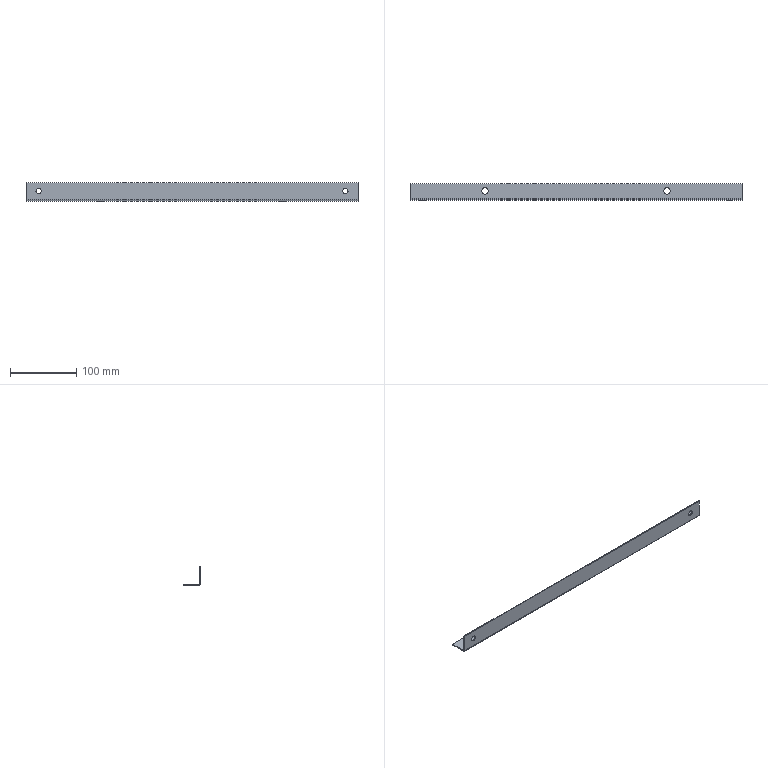Component | SolidWorks | ALK K_EBENT-3 | 1 solid | 22 faces | box 500 x 25.5 x 28.5 mm | volume 38510 mm3 | plane 12 | cylinder 10 | commonest cylinder face diameters 8 x4 10 x4 1.473 x1 4.473 x1
STEP:
#1=CARTESIAN_POINT('',(12.868,0.4007,-13.525));
#2=VERTEX_POINT('',#1);
#3=CARTESIAN_POINT('',(12.553,0.4007,-13.525));
#4=VERTEX_POINT('',#3);
#5=CARTESIAN_POINT('',(12.711,0.4007,-13.525));
#6=DIRECTION('',(0.,1.,0.));
#7=DIRECTION('',(-1.,0.,0.));
#8=AXIS2_PLACEMENT_3D('',#5,#6,#7);
#9=CIRCLE('',#8,0.1575);
#10=EDGE_CURVE('',#2,#4,#9,.T.);
#11=ORIENTED_EDGE('',*,*,#10,.F.);
#12=CARTESIAN_POINT('',(12.868,0.4597,-13.525));
#13=VERTEX_POINT('',#12);
#14=CARTESIAN_POINT('',(12.868,0.06603,-13.525));
#15=DIRECTION('',(0.,1.,0.));
#16=VECTOR('',#15,39.37);
#17=LINE('',#14,#16);
#18=EDGE_CURVE('',#2,#13,#17,.T.);
#19=ORIENTED_EDGE('',*,*,#18,.T.);
#20=CARTESIAN_POINT('',(12.553,0.4597,-13.525));
#21=VERTEX_POINT('',#20);
#22=CARTESIAN_POINT('',(12.711,0.4597,-13.525));
#23=DIRECTION('',(0.,1.,0.));
#24=DIRECTION('',(-1.,0.,0.));
#25=AXIS2_PLACEMENT_3D('',#22,#23,#24);
#26=CIRCLE('',#25,0.1575);
#27=EDGE_CURVE('',#13,#21,#26,.T.);
#28=ORIENTED_EDGE('',*,*,#27,.T.);
#29=CARTESIAN_POINT('',(12.553,0.06603,-13.525));
#30=DIRECTION('',(0.,1.,0.));
#31=VECTOR('',#30,39.37);
#32=LINE('',#29,#31);
#33=EDGE_CURVE('',#4,#21,#32,.T.);
#34=ORIENTED_EDGE('',*,*,#33,.F.);
#35=EDGE_LOOP('',(#11,#19,#28,#34));
#36=FACE_OUTER_BOUND('',#35,.T.);
#37=CARTESIAN_POINT('',(12.711,0.06603,-13.525));
#38=DIRECTION('',(0.,1.,0.));
#39=DIRECTION('',(-1.,0.,0.));
#40=AXIS2_PLACEMENT_3D('',#37,#38,#39);
#41=CYLINDRICAL_SURFACE('',#40,0.1575);
#42=ADVANCED_FACE('',(#36),#41,.F.);
#43=CARTESIAN_POINT('',(-5.321,0.4007,-13.525));
#44=VERTEX_POINT('',#43);
#45=CARTESIAN_POINT('',(-5.636,0.4007,-13.525));
#46=VERTEX_POINT('',#45);
#47=CARTESIAN_POINT('',(-5.478,0.4007,-13.525));
#48=DIRECTION('',(0.,1.,0.));
#49=DIRECTION('',(-1.,0.,0.));
#50=AXIS2_PLACEMENT_3D('',#47,#48,#49);
#51=CIRCLE('',#50,0.1575);
#52=EDGE_CURVE('',#44,#46,#51,.T.);
#53=ORIENTED_EDGE('',*,*,#52,.F.);
#54=CARTESIAN_POINT('',(-5.321,0.4597,-13.525));
#55=VERTEX_POINT('',#54);
#56=CARTESIAN_POINT('',(-5.321,0.06603,-13.525));
#57=DIRECTION('',(0.,1.,0.));
#58=VECTOR('',#57,39.37);
#59=LINE('',#56,#58);
#60=EDGE_CURVE('',#44,#55,#59,.T.);
#61=ORIENTED_EDGE('',*,*,#60,.T.);
#62=CARTESIAN_POINT('',(-5.636,0.4597,-13.525));
#63=VERTEX_POINT('',#62);
#64=CARTESIAN_POINT('',(-5.478,0.4597,-13.525));
#65=DIRECTION('',(0.,1.,0.));
#66=DIRECTION('',(-1.,0.,0.));
#67=AXIS2_PLACEMENT_3D('',#64,#65,#66);
#68=CIRCLE('',#67,0.1575);
#69=EDGE_CURVE('',#55,#63,#68,.T.);
#70=ORIENTED_EDGE('',*,*,#69,.T.);
#71=CARTESIAN_POINT('',(-5.636,0.06603,-13.525));
#72=DIRECTION('',(0.,1.,0.));
#73=VECTOR('',#72,39.37);
#74=LINE('',#71,#73);
#75=EDGE_CURVE('',#46,#63,#74,.T.);
#76=ORIENTED_EDGE('',*,*,#75,.F.);
#77=EDGE_LOOP('',(#53,#61,#70,#76));
#78=FACE_OUTER_BOUND('',#77,.T.);
#79=CARTESIAN_POINT('',(-5.478,0.06603,-13.525));
#80=DIRECTION('',(0.,1.,0.));
#81=DIRECTION('',(-1.,0.,0.));
#82=AXIS2_PLACEMENT_3D('',#79,#80,#81);
#83=CYLINDRICAL_SURFACE('',#82,0.1575);
#84=ADVANCED_FACE('',(#78),#83,.F.);
#85=CARTESIAN_POINT('',(8.813,0.9715,-14.076));
#86=VERTEX_POINT('',#85);
#87=CARTESIAN_POINT('',(9.207,0.9715,-14.076));
#88=VERTEX_POINT('',#87);
#89=CARTESIAN_POINT('',(9.01,0.9715,-14.076));
#90=DIRECTION('',(-0.,-0.,1.));
#91=DIRECTION('',(1.,0.,0.));
#92=AXIS2_PLACEMENT_3D('',#89,#90,#91);
#93=CIRCLE('',#92,0.1969);
#94=EDGE_CURVE('',#86,#88,#93,.T.);
#95=ORIENTED_EDGE('',*,*,#94,.T.);
#96=CARTESIAN_POINT('',(9.207,0.9715,-14.135));
#97=VERTEX_POINT('',#96);
#98=CARTESIAN_POINT('',(9.207,0.9715,-13.741));
#99=DIRECTION('',(0.,0.,-1.));
#100=VECTOR('',#99,39.37);
#101=LINE('',#98,#100);
#102=EDGE_CURVE('',#88,#97,#101,.T.);
#103=ORIENTED_EDGE('',*,*,#102,.T.);
#104=CARTESIAN_POINT('',(8.813,0.9715,-14.135));
#105=VERTEX_POINT('',#104);
#106=CARTESIAN_POINT('',(9.01,0.9715,-14.135));
#107=DIRECTION('',(0.,0.,-1.));
#108=DIRECTION('',(-1.,0.,0.));
#109=AXIS2_PLACEMENT_3D('',#106,#107,#108);
#110=CIRCLE('',#109,0.1969);
#111=EDGE_CURVE('',#97,#105,#110,.T.);
#112=ORIENTED_EDGE('',*,*,#111,.T.);
#113=CARTESIAN_POINT('',(8.813,0.9715,-13.741));
#114=DIRECTION('',(0.,0.,-1.));
#115=VECTOR('',#114,39.37);
#116=LINE('',#113,#115);
#117=EDGE_CURVE('',#86,#105,#116,.T.);
#118=ORIENTED_EDGE('',*,*,#117,.F.);
#119=EDGE_LOOP('',(#95,#103,#112,#118));
#120=FACE_OUTER_BOUND('',#119,.T.);
#121=CARTESIAN_POINT('',(9.01,0.9715,-13.741));
#122=DIRECTION('',(0.,0.,-1.));
#123=DIRECTION('',(-1.,0.,0.));
#124=AXIS2_PLACEMENT_3D('',#121,#122,#123);
#125=CYLINDRICAL_SURFACE('',#124,0.1969);
#126=ADVANCED_FACE('',(#120),#125,.F.);
#127=CARTESIAN_POINT('',(-1.974,0.9715,-14.076));
#128=VERTEX_POINT('',#127);
#129=CARTESIAN_POINT('',(-1.581,0.9715,-14.076));
#130=VERTEX_POINT('',#129);
#131=CARTESIAN_POINT('',(-1.777,0.9715,-14.076));
#132=DIRECTION('',(-0.,-0.,1.));
#133=DIRECTION('',(1.,0.,0.));
#134=AXIS2_PLACEMENT_3D('',#131,#132,#133);
#135=CIRCLE('',#134,0.1969);
#136=EDGE_CURVE('',#128,#130,#135,.T.);
#137=ORIENTED_EDGE('',*,*,#136,.T.);
#138=CARTESIAN_POINT('',(-1.581,0.9715,-14.135));
#139=VERTEX_POINT('',#138);
#140=CARTESIAN_POINT('',(-1.581,0.9715,-13.741));
#141=DIRECTION('',(0.,0.,-1.));
#142=VECTOR('',#141,39.37);
#143=LINE('',#140,#142);
#144=EDGE_CURVE('',#130,#139,#143,.T.);
#145=ORIENTED_EDGE('',*,*,#144,.T.);
#146=CARTESIAN_POINT('',(-1.974,0.9715,-14.135));
#147=VERTEX_POINT('',#146);
#148=CARTESIAN_POINT('',(-1.777,0.9715,-14.135));
#149=DIRECTION('',(0.,0.,-1.));
#150=DIRECTION('',(-1.,0.,0.));
#151=AXIS2_PLACEMENT_3D('',#148,#149,#150);
#152=CIRCLE('',#151,0.1969);
#153=EDGE_CURVE('',#139,#147,#152,.T.);
#154=ORIENTED_EDGE('',*,*,#153,.T.);
#155=CARTESIAN_POINT('',(-1.974,0.9715,-13.741));
#156=DIRECTION('',(0.,0.,-1.));
#157=VECTOR('',#156,39.37);
#158=LINE('',#155,#157);
#159=EDGE_CURVE('',#128,#147,#158,.T.);
#160=ORIENTED_EDGE('',*,*,#159,.F.);
#161=EDGE_LOOP('',(#137,#145,#154,#160));
#162=FACE_OUTER_BOUND('',#161,.T.);
#163=CARTESIAN_POINT('',(-1.777,0.9715,-13.741));
#164=DIRECTION('',(0.,0.,-1.));
#165=DIRECTION('',(-1.,0.,0.));
#166=AXIS2_PLACEMENT_3D('',#163,#164,#165);
#167=CYLINDRICAL_SURFACE('',#166,0.1969);
#168=ADVANCED_FACE('',(#162),#167,.F.);
#169=CARTESIAN_POINT('',(-6.226,0.4597,-14.047));
#170=VERTEX_POINT('',#169);
#171=CARTESIAN_POINT('',(-6.226,0.4007,-14.047));
#172=VERTEX_POINT('',#171);
#173=CARTESIAN_POINT('',(-6.226,0.4597,-14.047));
#174=DIRECTION('',(-0.,-1.,-0.));
#175=VECTOR('',#174,39.37);
#176=LINE('',#173,#175);
#177=EDGE_CURVE('',#170,#172,#176,.T.);
#178=ORIENTED_EDGE('',*,*,#177,.F.);
#179=CARTESIAN_POINT('',(-6.226,0.4887,-14.076));
#180=VERTEX_POINT('',#179);
#181=CARTESIAN_POINT('',(-6.226,0.4887,-14.047));
#182=DIRECTION('',(-1.,0.,-0.));
#183=DIRECTION('',(0.,0.,-1.));
#184=AXIS2_PLACEMENT_3D('',#181,#182,#183);
#185=CIRCLE('',#184,0.029);
#186=EDGE_CURVE('',#180,#170,#185,.T.);
#187=ORIENTED_EDGE('',*,*,#186,.F.);
#188=CARTESIAN_POINT('',(-6.226,0.4887,-14.135));
#189=VERTEX_POINT('',#188);
#190=CARTESIAN_POINT('',(-6.226,0.4887,-14.135));
#191=DIRECTION('',(-0.,-0.,1.));
#192=VECTOR('',#191,39.37);
#193=LINE('',#190,#192);
#194=EDGE_CURVE('',#189,#180,#193,.T.);
#195=ORIENTED_EDGE('',*,*,#194,.F.);
#196=CARTESIAN_POINT('',(-6.226,0.4887,-14.047));
#197=DIRECTION('',(-1.,0.,-0.));
#198=DIRECTION('',(0.,0.,1.));
#199=AXIS2_PLACEMENT_3D('',#196,#197,#198);
#200=CIRCLE('',#199,0.08806);
#201=EDGE_CURVE('',#189,#172,#200,.T.);
#202=ORIENTED_EDGE('',*,*,#201,.T.);
#203=EDGE_LOOP('',(#178,#187,#195,#202));
#204=FACE_OUTER_BOUND('',#203,.T.);
#205=CARTESIAN_POINT('',(-6.226,0.4597,-14.047));
#206=DIRECTION('',(-1.,0.,-0.));
#207=DIRECTION('',(-0.,-0.,1.));
#208=AXIS2_PLACEMENT_3D('',#205,#206,#207);
#209=PLANE('',#208);
#210=ADVANCED_FACE('',(#204),#209,.T.);
#211=CARTESIAN_POINT('',(-6.226,0.4597,-13.013));
#212=VERTEX_POINT('',#211);
#213=CARTESIAN_POINT('',(-6.226,0.4597,-14.076));
#214=DIRECTION('',(-0.,-0.,1.));
#215=VECTOR('',#214,39.37);
#216=LINE('',#213,#215);
#217=EDGE_CURVE('',#170,#212,#216,.T.);
#218=ORIENTED_EDGE('',*,*,#217,.F.);
#219=ORIENTED_EDGE('',*,*,#177,.T.);
#220=CARTESIAN_POINT('',(-6.226,0.4007,-13.013));
#221=VERTEX_POINT('',#220);
#222=CARTESIAN_POINT('',(-6.226,0.4007,-14.076));
#223=DIRECTION('',(-0.,-0.,1.));
#224=VECTOR('',#223,39.37);
#225=LINE('',#222,#224);
#226=EDGE_CURVE('',#172,#221,#225,.T.);
#227=ORIENTED_EDGE('',*,*,#226,.T.);
#228=CARTESIAN_POINT('',(-6.226,0.4597,-13.013));
#229=DIRECTION('',(-0.,-1.,-0.));
#230=VECTOR('',#229,39.37);
#231=LINE('',#228,#230);
#232=EDGE_CURVE('',#212,#221,#231,.T.);
#233=ORIENTED_EDGE('',*,*,#232,.F.);
#234=EDGE_LOOP('',(#218,#219,#227,#233));
#235=FACE_OUTER_BOUND('',#234,.T.);
#236=CARTESIAN_POINT('',(-6.226,0.4887,-14.135));
#237=DIRECTION('',(-1.,0.,-0.));
#238=DIRECTION('',(-0.,-0.,1.));
#239=AXIS2_PLACEMENT_3D('',#236,#237,#238);
#240=PLANE('',#239);
#241=ADVANCED_FACE('',(#235),#240,.T.);
#242=CARTESIAN_POINT('',(13.459,0.4887,-14.076));
#243=VERTEX_POINT('',#242);
#244=CARTESIAN_POINT('',(13.459,0.4887,-14.135));
#245=VERTEX_POINT('',#244);
#246=CARTESIAN_POINT('',(13.459,0.4887,-14.076));
#247=DIRECTION('',(0.,0.,-1.));
#248=VECTOR('',#247,39.37);
#249=LINE('',#246,#248);
#250=EDGE_CURVE('',#243,#245,#249,.T.);
#251=ORIENTED_EDGE('',*,*,#250,.F.);
#252=CARTESIAN_POINT('',(13.459,0.4597,-14.047));
#253=VERTEX_POINT('',#252);
#254=CARTESIAN_POINT('',(13.459,0.4887,-14.047));
#255=DIRECTION('',(-1.,0.,-0.));
#256=DIRECTION('',(0.,0.,-1.));
#257=AXIS2_PLACEMENT_3D('',#254,#255,#256);
#258=CIRCLE('',#257,0.029);
#259=EDGE_CURVE('',#243,#253,#258,.T.);
#260=ORIENTED_EDGE('',*,*,#259,.T.);
#261=CARTESIAN_POINT('',(13.459,0.4007,-14.047));
#262=VERTEX_POINT('',#261);
#263=CARTESIAN_POINT('',(13.459,0.4007,-14.047));
#264=DIRECTION('',(0.,1.,0.));
#265=VECTOR('',#264,39.37);
#266=LINE('',#263,#265);
#267=EDGE_CURVE('',#262,#253,#266,.T.);
#268=ORIENTED_EDGE('',*,*,#267,.F.);
#269=CARTESIAN_POINT('',(13.459,0.4887,-14.047));
#270=DIRECTION('',(-1.,0.,-0.));
#271=DIRECTION('',(0.,0.,1.));
#272=AXIS2_PLACEMENT_3D('',#269,#270,#271);
#273=CIRCLE('',#272,0.08806);
#274=EDGE_CURVE('',#245,#262,#273,.T.);
#275=ORIENTED_EDGE('',*,*,#274,.F.);
#276=EDGE_LOOP('',(#251,#260,#268,#275));
#277=FACE_OUTER_BOUND('',#276,.T.);
#278=CARTESIAN_POINT('',(13.459,0.4887,-14.076));
#279=DIRECTION('',(1.,-0.,0.));
#280=DIRECTION('',(0.,0.,-1.));
#281=AXIS2_PLACEMENT_3D('',#278,#279,#280);
#282=PLANE('',#281);
#283=ADVANCED_FACE('',(#277),#282,.T.);
#284=CARTESIAN_POINT('',(13.459,1.405,-14.076));
#285=VERTEX_POINT('',#284);
#286=CARTESIAN_POINT('',(13.459,0.4597,-14.076));
#287=DIRECTION('',(-0.,-1.,-0.));
#288=VECTOR('',#287,39.37);
#289=LINE('',#286,#288);
#290=EDGE_CURVE('',#285,#243,#289,.T.);
#291=ORIENTED_EDGE('',*,*,#290,.T.);
#292=ORIENTED_EDGE('',*,*,#250,.T.);
#293=CARTESIAN_POINT('',(13.459,1.405,-14.135));
#294=VERTEX_POINT('',#293);
#295=CARTESIAN_POINT('',(13.459,0.4597,-14.135));
#296=DIRECTION('',(-0.,-1.,-0.));
#297=VECTOR('',#296,39.37);
#298=LINE('',#295,#297);
#299=EDGE_CURVE('',#294,#245,#298,.T.);
#300=ORIENTED_EDGE('',*,*,#299,.F.);
#301=CARTESIAN_POINT('',(13.459,1.405,-14.135));
#302=DIRECTION('',(-0.,-0.,1.));
#303=VECTOR('',#302,39.37);
#304=LINE('',#301,#303);
#305=EDGE_CURVE('',#294,#285,#304,.T.);
#306=ORIENTED_EDGE('',*,*,#305,.T.);
#307=EDGE_LOOP('',(#291,#292,#300,#306));
#308=FACE_OUTER_BOUND('',#307,.T.);
#309=CARTESIAN_POINT('',(13.459,0.4007,-14.047));
#310=DIRECTION('',(1.,-0.,0.));
#311=DIRECTION('',(0.,0.,-1.));
#312=AXIS2_PLACEMENT_3D('',#309,#310,#311);
#313=PLANE('',#312);
#314=ADVANCED_FACE('',(#308),#313,.T.);
#315=CARTESIAN_POINT('',(12.711,0.4007,-13.525));
#316=DIRECTION('',(0.,1.,0.));
#317=DIRECTION('',(-1.,0.,0.));
#318=AXIS2_PLACEMENT_3D('',#315,#316,#317);
#319=CIRCLE('',#318,0.1575);
#320=EDGE_CURVE('',#4,#2,#319,.T.);
#321=ORIENTED_EDGE('',*,*,#320,.T.);
#322=ORIENTED_EDGE('',*,*,#10,.T.);
#323=EDGE_LOOP('',(#321,#322));
#324=FACE_BOUND('',#323,.T.);
#325=CARTESIAN_POINT('',(-5.478,0.4007,-13.525));
#326=DIRECTION('',(0.,1.,0.));
#327=DIRECTION('',(-1.,0.,0.));
#328=AXIS2_PLACEMENT_3D('',#325,#326,#327);
#329=CIRCLE('',#328,0.1575);
#330=EDGE_CURVE('',#46,#44,#329,.T.);
#331=ORIENTED_EDGE('',*,*,#330,.T.);
#332=ORIENTED_EDGE('',*,*,#52,.T.);
#333=EDGE_LOOP('',(#331,#332));
#334=FACE_BOUND('',#333,.T.);
#335=CARTESIAN_POINT('',(13.459,0.4007,-13.013));
#336=VERTEX_POINT('',#335);
#337=CARTESIAN_POINT('',(13.459,0.4007,-14.076));
#338=DIRECTION('',(-0.,-0.,1.));
#339=VECTOR('',#338,39.37);
#340=LINE('',#337,#339);
#341=EDGE_CURVE('',#262,#336,#340,.T.);
#342=ORIENTED_EDGE('',*,*,#341,.T.);
#343=CARTESIAN_POINT('',(-6.226,0.4007,-13.013));
#344=DIRECTION('',(1.,-0.,0.));
#345=VECTOR('',#344,39.37);
#346=LINE('',#343,#345);
#347=EDGE_CURVE('',#221,#336,#346,.T.);
#348=ORIENTED_EDGE('',*,*,#347,.F.);
#349=ORIENTED_EDGE('',*,*,#226,.F.);
#350=CARTESIAN_POINT('',(-6.226,0.4007,-14.047));
#351=DIRECTION('',(1.,-0.,0.));
#352=VECTOR('',#351,39.37);
#353=LINE('',#350,#352);
#354=EDGE_CURVE('',#172,#262,#353,.T.);
#355=ORIENTED_EDGE('',*,*,#354,.T.);
#356=EDGE_LOOP('',(#342,#348,#349,#355));
#357=FACE_OUTER_BOUND('',#356,.T.);
#358=CARTESIAN_POINT('',(-6.226,0.4007,-14.076));
#359=DIRECTION('',(0.,1.,0.));
#360=DIRECTION('',(-1.,0.,-0.));
#361=AXIS2_PLACEMENT_3D('',#358,#359,#360);
#362=PLANE('',#361);
#363=ADVANCED_FACE('',(#324,#334,#357),#362,.F.);
#364=CARTESIAN_POINT('',(13.459,0.4597,-13.013));
#365=VERTEX_POINT('',#364);
#366=CARTESIAN_POINT('',(13.459,0.4597,-13.013));
#367=DIRECTION('',(-0.,-1.,-0.));
#368=VECTOR('',#367,39.37);
#369=LINE('',#366,#368);
#370=EDGE_CURVE('',#365,#336,#369,.T.);
#371=ORIENTED_EDGE('',*,*,#370,.F.);
#372=CARTESIAN_POINT('',(-6.226,0.4597,-13.013));
#373=DIRECTION('',(1.,-0.,0.));
#374=VECTOR('',#373,39.37);
#375=LINE('',#372,#374);
#376=EDGE_CURVE('',#212,#365,#375,.T.);
#377=ORIENTED_EDGE('',*,*,#376,.F.);
#378=ORIENTED_EDGE('',*,*,#232,.T.);
#379=ORIENTED_EDGE('',*,*,#347,.T.);
#380=EDGE_LOOP('',(#371,#377,#378,#379));
#381=FACE_OUTER_BOUND('',#380,.T.);
#382=CARTESIAN_POINT('',(-6.226,0.4597,-13.013));
#383=DIRECTION('',(-0.,-0.,1.));
#384=DIRECTION('',(1.,-0.,0.));
#385=AXIS2_PLACEMENT_3D('',#382,#383,#384);
#386=PLANE('',#385);
#387=ADVANCED_FACE('',(#381),#386,.T.);
#388=CARTESIAN_POINT('',(12.711,0.4597,-13.525));
#389=DIRECTION('',(0.,1.,0.));
#390=DIRECTION('',(-1.,0.,0.));
#391=AXIS2_PLACEMENT_3D('',#388,#389,#390);
#392=CIRCLE('',#391,0.1575);
#393=EDGE_CURVE('',#21,#13,#392,.T.);
#394=ORIENTED_EDGE('',*,*,#393,.F.);
#395=ORIENTED_EDGE('',*,*,#27,.F.);
#396=EDGE_LOOP('',(#394,#395));
#397=FACE_BOUND('',#396,.T.);
#398=CARTESIAN_POINT('',(-5.478,0.4597,-13.525));
#399=DIRECTION('',(0.,1.,0.));
#400=DIRECTION('',(-1.,0.,0.));
#401=AXIS2_PLACEMENT_3D('',#398,#399,#400);
#402=CIRCLE('',#401,0.1575);
#403=EDGE_CURVE('',#63,#55,#402,.T.);
#404=ORIENTED_EDGE('',*,*,#403,.F.);
#405=ORIENTED_EDGE('',*,*,#69,.F.);
#406=EDGE_LOOP('',(#404,#405));
#407=FACE_BOUND('',#406,.T.);
#408=CARTESIAN_POINT('',(13.459,0.4597,-14.076));
#409=DIRECTION('',(-0.,-0.,1.));
#410=VECTOR('',#409,39.37);
#411=LINE('',#408,#410);
#412=EDGE_CURVE('',#253,#365,#411,.T.);
#413=ORIENTED_EDGE('',*,*,#412,.F.);
#414=CARTESIAN_POINT('',(-6.226,0.4597,-14.047));
#415=DIRECTION('',(1.,-0.,0.));
#416=VECTOR('',#415,39.37);
#417=LINE('',#414,#416);
#418=EDGE_CURVE('',#170,#253,#417,.T.);
#419=ORIENTED_EDGE('',*,*,#418,.F.);
#420=ORIENTED_EDGE('',*,*,#217,.T.);
#421=ORIENTED_EDGE('',*,*,#376,.T.);
#422=EDGE_LOOP('',(#413,#419,#420,#421));
#423=FACE_OUTER_BOUND('',#422,.T.);
#424=CARTESIAN_POINT('',(-6.226,0.4597,-14.076));
#425=DIRECTION('',(0.,1.,0.));
#426=DIRECTION('',(-1.,0.,-0.));
#427=AXIS2_PLACEMENT_3D('',#424,#425,#426);
#428=PLANE('',#427);
#429=ADVANCED_FACE('',(#397,#407,#423),#428,.T.);
#430=ORIENTED_EDGE('',*,*,#259,.F.);
#431=CARTESIAN_POINT('',(-6.226,0.4887,-14.076));
#432=DIRECTION('',(1.,-0.,0.));
#433=VECTOR('',#432,39.37);
#434=LINE('',#431,#433);
#435=EDGE_CURVE('',#180,#243,#434,.T.);
#436=ORIENTED_EDGE('',*,*,#435,.F.);
#437=ORIENTED_EDGE('',*,*,#186,.T.);
#438=ORIENTED_EDGE('',*,*,#418,.T.);
#439=EDGE_LOOP('',(#430,#436,#437,#438));
#440=FACE_OUTER_BOUND('',#439,.T.);
#441=CARTESIAN_POINT('',(-6.226,0.4887,-14.047));
#442=DIRECTION('',(1.,-0.,0.));
#443=DIRECTION('',(0.,0.,-1.));
#444=AXIS2_PLACEMENT_3D('',#441,#442,#443);
#445=CYLINDRICAL_SURFACE('',#444,0.029);
#446=ADVANCED_FACE('',(#440),#445,.F.);
#447=ORIENTED_EDGE('',*,*,#94,.F.);
#448=CARTESIAN_POINT('',(9.01,0.9715,-14.076));
#449=DIRECTION('',(-0.,-0.,1.));
#450=DIRECTION('',(1.,0.,0.));
#451=AXIS2_PLACEMENT_3D('',#448,#449,#450);
#452=CIRCLE('',#451,0.1969);
#453=EDGE_CURVE('',#88,#86,#452,.T.);
#454=ORIENTED_EDGE('',*,*,#453,.F.);
#455=EDGE_LOOP('',(#447,#454));
#456=FACE_BOUND('',#455,.T.);
#457=ORIENTED_EDGE('',*,*,#136,.F.);
#458=CARTESIAN_POINT('',(-1.777,0.9715,-14.076));
#459=DIRECTION('',(-0.,-0.,1.));
#460=DIRECTION('',(1.,0.,0.));
#461=AXIS2_PLACEMENT_3D('',#458,#459,#460);
#462=CIRCLE('',#461,0.1969);
#463=EDGE_CURVE('',#130,#128,#462,.T.);
#464=ORIENTED_EDGE('',*,*,#463,.F.);
#465=EDGE_LOOP('',(#457,#464));
#466=FACE_BOUND('',#465,.T.);
#467=ORIENTED_EDGE('',*,*,#290,.F.);
#468=CARTESIAN_POINT('',(-6.226,1.405,-14.076));
#469=VERTEX_POINT('',#468);
#470=CARTESIAN_POINT('',(-6.226,1.405,-14.076));
#471=DIRECTION('',(1.,-0.,0.));
#472=VECTOR('',#471,39.37);
#473=LINE('',#470,#472);
#474=EDGE_CURVE('',#469,#285,#473,.T.);
#475=ORIENTED_EDGE('',*,*,#474,.F.);
#476=CARTESIAN_POINT('',(-6.226,0.4597,-14.076));
#477=DIRECTION('',(-0.,-1.,-0.));
#478=VECTOR('',#477,39.37);
#479=LINE('',#476,#478);
#480=EDGE_CURVE('',#469,#180,#479,.T.);
#481=ORIENTED_EDGE('',*,*,#480,.T.);
#482=ORIENTED_EDGE('',*,*,#435,.T.);
#483=EDGE_LOOP('',(#467,#475,#481,#482));
#484=FACE_OUTER_BOUND('',#483,.T.);
#485=CARTESIAN_POINT('',(-6.226,0.4597,-14.076));
#486=DIRECTION('',(-0.,-0.,1.));
#487=DIRECTION('',(1.,-0.,0.));
#488=AXIS2_PLACEMENT_3D('',#485,#486,#487);
#489=PLANE('',#488);
#490=ADVANCED_FACE('',(#456,#466,#484),#489,.T.);
#491=ORIENTED_EDGE('',*,*,#305,.F.);
#492=CARTESIAN_POINT('',(-6.226,1.405,-14.135));
#493=VERTEX_POINT('',#492);
#494=CARTESIAN_POINT('',(-6.226,1.405,-14.135));
#495=DIRECTION('',(1.,-0.,0.));
#496=VECTOR('',#495,39.37);
#497=LINE('',#494,#496);
#498=EDGE_CURVE('',#493,#294,#497,.T.);
#499=ORIENTED_EDGE('',*,*,#498,.F.);
#500=CARTESIAN_POINT('',(-6.226,1.405,-14.135));
#501=DIRECTION('',(-0.,-0.,1.));
#502=VECTOR('',#501,39.37);
#503=LINE('',#500,#502);
#504=EDGE_CURVE('',#493,#469,#503,.T.);
#505=ORIENTED_EDGE('',*,*,#504,.T.);
#506=ORIENTED_EDGE('',*,*,#474,.T.);
#507=EDGE_LOOP('',(#491,#499,#505,#506));
#508=FACE_OUTER_BOUND('',#507,.T.);
#509=CARTESIAN_POINT('',(-6.226,1.405,-14.135));
#510=DIRECTION('',(0.,1.,0.));
#511=DIRECTION('',(-1.,0.,-0.));
#512=AXIS2_PLACEMENT_3D('',#509,#510,#511);
#513=PLANE('',#512);
#514=ADVANCED_FACE('',(#508),#513,.T.);
#515=CARTESIAN_POINT('',(9.01,0.9715,-14.135));
#516=DIRECTION('',(0.,0.,-1.));
#517=DIRECTION('',(-1.,0.,0.));
#518=AXIS2_PLACEMENT_3D('',#515,#516,#517);
#519=CIRCLE('',#518,0.1969);
#520=EDGE_CURVE('',#105,#97,#519,.T.);
#521=ORIENTED_EDGE('',*,*,#520,.F.);
#522=ORIENTED_EDGE('',*,*,#111,.F.);
#523=EDGE_LOOP('',(#521,#522));
#524=FACE_BOUND('',#523,.T.);
#525=CARTESIAN_POINT('',(-1.777,0.9715,-14.135));
#526=DIRECTION('',(0.,0.,-1.));
#527=DIRECTION('',(-1.,0.,0.));
#528=AXIS2_PLACEMENT_3D('',#525,#526,#527);
#529=CIRCLE('',#528,0.1969);
#530=EDGE_CURVE('',#147,#139,#529,.T.);
#531=ORIENTED_EDGE('',*,*,#530,.F.);
#532=ORIENTED_EDGE('',*,*,#153,.F.);
#533=EDGE_LOOP('',(#531,#532));
#534=FACE_BOUND('',#533,.T.);
#535=ORIENTED_EDGE('',*,*,#299,.T.);
#536=CARTESIAN_POINT('',(-6.226,0.4887,-14.135));
#537=DIRECTION('',(1.,-0.,0.));
#538=VECTOR('',#537,39.37);
#539=LINE('',#536,#538);
#540=EDGE_CURVE('',#189,#245,#539,.T.);
#541=ORIENTED_EDGE('',*,*,#540,.F.);
#542=CARTESIAN_POINT('',(-6.226,0.4597,-14.135));
#543=DIRECTION('',(-0.,-1.,-0.));
#544=VECTOR('',#543,39.37);
#545=LINE('',#542,#544);
#546=EDGE_CURVE('',#493,#189,#545,.T.);
#547=ORIENTED_EDGE('',*,*,#546,.F.);
#548=ORIENTED_EDGE('',*,*,#498,.T.);
#549=EDGE_LOOP('',(#535,#541,#547,#548));
#550=FACE_OUTER_BOUND('',#549,.T.);
#551=CARTESIAN_POINT('',(-6.226,0.4597,-14.135));
#552=DIRECTION('',(-0.,-0.,1.));
#553=DIRECTION('',(1.,-0.,0.));
#554=AXIS2_PLACEMENT_3D('',#551,#552,#553);
#555=PLANE('',#554);
#556=ADVANCED_FACE('',(#524,#534,#550),#555,.F.);
#557=ORIENTED_EDGE('',*,*,#274,.T.);
#558=ORIENTED_EDGE('',*,*,#354,.F.);
#559=ORIENTED_EDGE('',*,*,#201,.F.);
#560=ORIENTED_EDGE('',*,*,#540,.T.);
#561=EDGE_LOOP('',(#557,#558,#559,#560));
#562=FACE_OUTER_BOUND('',#561,.T.);
#563=CARTESIAN_POINT('',(-6.226,0.4887,-14.047));
#564=DIRECTION('',(1.,-0.,0.));
#565=DIRECTION('',(0.,0.,-1.));
#566=AXIS2_PLACEMENT_3D('',#563,#564,#565);
#567=CYLINDRICAL_SURFACE('',#566,0.08806);
#568=ADVANCED_FACE('',(#562),#567,.T.);
#569=ORIENTED_EDGE('',*,*,#546,.T.);
#570=ORIENTED_EDGE('',*,*,#194,.T.);
#571=ORIENTED_EDGE('',*,*,#480,.F.);
#572=ORIENTED_EDGE('',*,*,#504,.F.);
#573=EDGE_LOOP('',(#569,#570,#571,#572));
#574=FACE_OUTER_BOUND('',#573,.T.);
#575=CARTESIAN_POINT('',(-6.226,0.4887,-14.047));
#576=DIRECTION('',(1.,-0.,0.));
#577=DIRECTION('',(0.,0.,-1.));
#578=AXIS2_PLACEMENT_3D('',#575,#576,#577);
#579=PLANE('',#578);
#580=ADVANCED_FACE('',(#574),#579,.F.);
#581=ORIENTED_EDGE('',*,*,#341,.F.);
#582=ORIENTED_EDGE('',*,*,#267,.T.);
#583=ORIENTED_EDGE('',*,*,#412,.T.);
#584=ORIENTED_EDGE('',*,*,#370,.T.);
#585=EDGE_LOOP('',(#581,#582,#583,#584));
#586=FACE_OUTER_BOUND('',#585,.T.);
#587=CARTESIAN_POINT('',(13.459,0.4887,-14.047));
#588=DIRECTION('',(1.,-0.,0.));
#589=DIRECTION('',(0.,0.,-1.));
#590=AXIS2_PLACEMENT_3D('',#587,#588,#589);
#591=PLANE('',#590);
#592=ADVANCED_FACE('',(#586),#591,.T.);
#593=ORIENTED_EDGE('',*,*,#144,.F.);
#594=ORIENTED_EDGE('',*,*,#463,.T.);
#595=ORIENTED_EDGE('',*,*,#159,.T.);
#596=ORIENTED_EDGE('',*,*,#530,.T.);
#597=EDGE_LOOP('',(#593,#594,#595,#596));
#598=FACE_OUTER_BOUND('',#597,.T.);
#599=CARTESIAN_POINT('',(-1.777,0.9715,-13.741));
#600=DIRECTION('',(0.,0.,-1.));
#601=DIRECTION('',(-1.,0.,0.));
#602=AXIS2_PLACEMENT_3D('',#599,#600,#601);
#603=CYLINDRICAL_SURFACE('',#602,0.1969);
#604=ADVANCED_FACE('',(#598),#603,.F.);
#605=ORIENTED_EDGE('',*,*,#102,.F.);
#606=ORIENTED_EDGE('',*,*,#453,.T.);
#607=ORIENTED_EDGE('',*,*,#117,.T.);
#608=ORIENTED_EDGE('',*,*,#520,.T.);
#609=EDGE_LOOP('',(#605,#606,#607,#608));
#610=FACE_OUTER_BOUND('',#609,.T.);
#611=CARTESIAN_POINT('',(9.01,0.9715,-13.741));
#612=DIRECTION('',(0.,0.,-1.));
#613=DIRECTION('',(-1.,0.,0.));
#614=AXIS2_PLACEMENT_3D('',#611,#612,#613);
#615=CYLINDRICAL_SURFACE('',#614,0.1969);
#616=ADVANCED_FACE('',(#610),#615,.F.);
#617=ORIENTED_EDGE('',*,*,#60,.F.);
#618=ORIENTED_EDGE('',*,*,#330,.F.);
#619=ORIENTED_EDGE('',*,*,#75,.T.);
#620=ORIENTED_EDGE('',*,*,#403,.T.);
#621=EDGE_LOOP('',(#617,#618,#619,#620));
#622=FACE_OUTER_BOUND('',#621,.T.);
#623=CARTESIAN_POINT('',(-5.478,0.06603,-13.525));
#624=DIRECTION('',(0.,1.,0.));
#625=DIRECTION('',(-1.,0.,0.));
#626=AXIS2_PLACEMENT_3D('',#623,#624,#625);
#627=CYLINDRICAL_SURFACE('',#626,0.1575);
#628=ADVANCED_FACE('',(#622),#627,.F.);
#629=ORIENTED_EDGE('',*,*,#18,.F.);
#630=ORIENTED_EDGE('',*,*,#320,.F.);
#631=ORIENTED_EDGE('',*,*,#33,.T.);
#632=ORIENTED_EDGE('',*,*,#393,.T.);
#633=EDGE_LOOP('',(#629,#630,#631,#632));
#634=FACE_OUTER_BOUND('',#633,.T.);
#635=CARTESIAN_POINT('',(12.711,0.06603,-13.525));
#636=DIRECTION('',(0.,1.,0.));
#637=DIRECTION('',(-1.,0.,0.));
#638=AXIS2_PLACEMENT_3D('',#635,#636,#637);
#639=CYLINDRICAL_SURFACE('',#638,0.1575);
#640=ADVANCED_FACE('',(#634),#639,.F.);
#641=CLOSED_SHELL('',(#42,#84,#126,#168,#210,#241,#283,#314,#363,#387,#429,#446,#490,#514,#556,#568,#580,#592,#604,#616,#628,#640));
#642=MANIFOLD_SOLID_BREP('',#641);
#643=CARTESIAN_POINT('',(0.,0.,0.));
#644=DIRECTION('',(0.,0.,1.));
#645=DIRECTION('',(1.,0.,0.));
#646=AXIS2_PLACEMENT_3D('',#643,#644,#645);
#647=(LENGTH_UNIT()NAMED_UNIT(*)SI_UNIT($,.METRE.));
#648=LENGTH_MEASURE_WITH_UNIT(LENGTH_MEASURE(0.0254),#647);
#649=DIMENSIONAL_EXPONENTS(1.,0.,0.,0.,0.,0.,0.);
#650=(CONVERSION_BASED_UNIT('',#648)LENGTH_UNIT()NAMED_UNIT(#649));
#651=UNCERTAINTY_MEASURE_WITH_UNIT(LENGTH_MEASURE(0.00001),#650,'','');
#652=(NAMED_UNIT(*)PLANE_ANGLE_UNIT()SI_UNIT($,.RADIAN.));
#653=(NAMED_UNIT(*)SI_UNIT($,.STERADIAN.)SOLID_ANGLE_UNIT());
#654=(GEOMETRIC_REPRESENTATION_CONTEXT(3)GLOBAL_UNCERTAINTY_ASSIGNED_CONTEXT((#651))GLOBAL_UNIT_ASSIGNED_CONTEXT((#650,#652,#653))REPRESENTATION_CONTEXT('',''));
#655=ADVANCED_BREP_SHAPE_REPRESENTATION('',(#642,#646),#654);
#656=COLOUR_RGB('',0.7922,0.8196,0.9333);
#657=FILL_AREA_STYLE_COLOUR('',#656);
#658=FILL_AREA_STYLE('',(#657));
#659=SURFACE_STYLE_FILL_AREA(#658);
#660=SURFACE_SIDE_STYLE('',(#659));
#661=SURFACE_STYLE_USAGE(.BOTH.,#660);
#662=PRESENTATION_STYLE_ASSIGNMENT((#661));
#663=STYLED_ITEM('',(#662),#642);
#664=PRESENTATION_LAYER_ASSIGNMENT('','',(#663));
#665=(LENGTH_UNIT()NAMED_UNIT(*)SI_UNIT($,.METRE.));
#666=LENGTH_MEASURE_WITH_UNIT(LENGTH_MEASURE(0.0254),#665);
#667=DIMENSIONAL_EXPONENTS(1.,0.,0.,0.,0.,0.,0.);
#668=(CONVERSION_BASED_UNIT('',#666)LENGTH_UNIT()NAMED_UNIT(#667));
#669=UNCERTAINTY_MEASURE_WITH_UNIT(LENGTH_MEASURE(0.00001),#668,'','');
#670=(NAMED_UNIT(*)PLANE_ANGLE_UNIT()SI_UNIT($,.RADIAN.));
#671=(NAMED_UNIT(*)SI_UNIT($,.STERADIAN.)SOLID_ANGLE_UNIT());
#672=(GEOMETRIC_REPRESENTATION_CONTEXT(3)GLOBAL_UNCERTAINTY_ASSIGNED_CONTEXT((#669))GLOBAL_UNIT_ASSIGNED_CONTEXT((#668,#670,#671))REPRESENTATION_CONTEXT('',''));
#673=MECHANICAL_DESIGN_GEOMETRIC_PRESENTATION_REPRESENTATION('',(#663),#672);